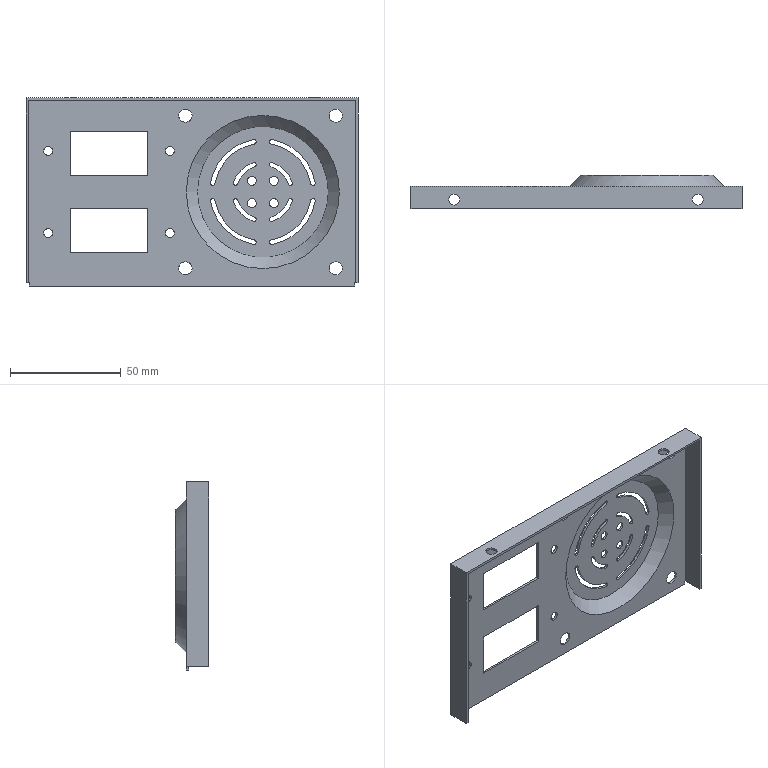Component | NX | FRONT_PANEL | 1 solid | 72 faces | volume 14000 mm3 | cylinder 46 | plane 24 | cone 2 | commonest cylinder face diameters 2 x16 4 x8 44 x4 48 x4 24 x4 28 x4 6 x4 5 x2